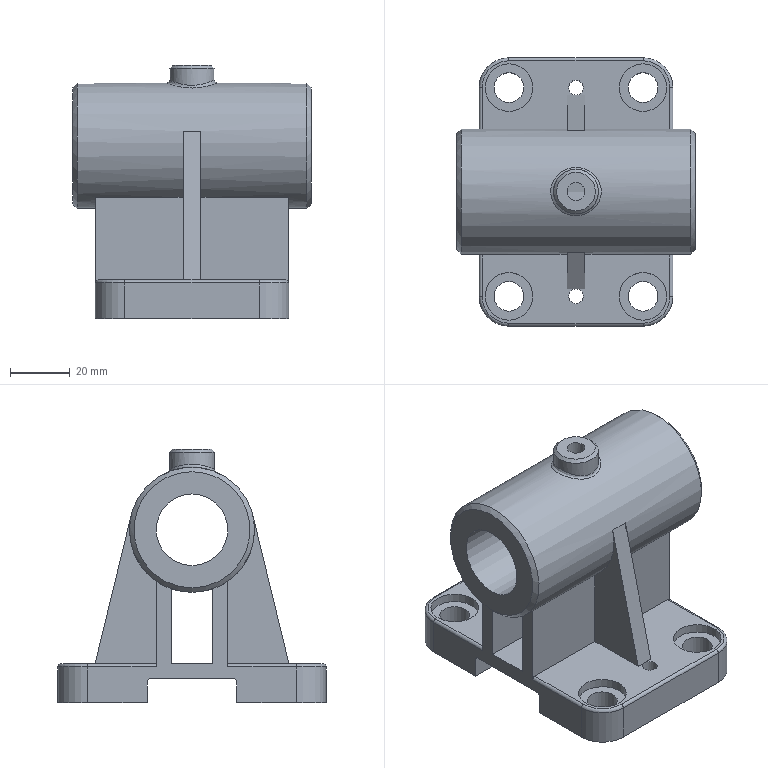Component | NX | BRACKET | 1 solid | 79 faces | volume 144102 mm3 | plane 33 | cylinder 32 | cone 7 | torus 6 | spline 1 | commonest cylinder face diameters 2 x8 4 x4 10 x4 16 x4 20 x4 24 x2 5 x2 42 x1